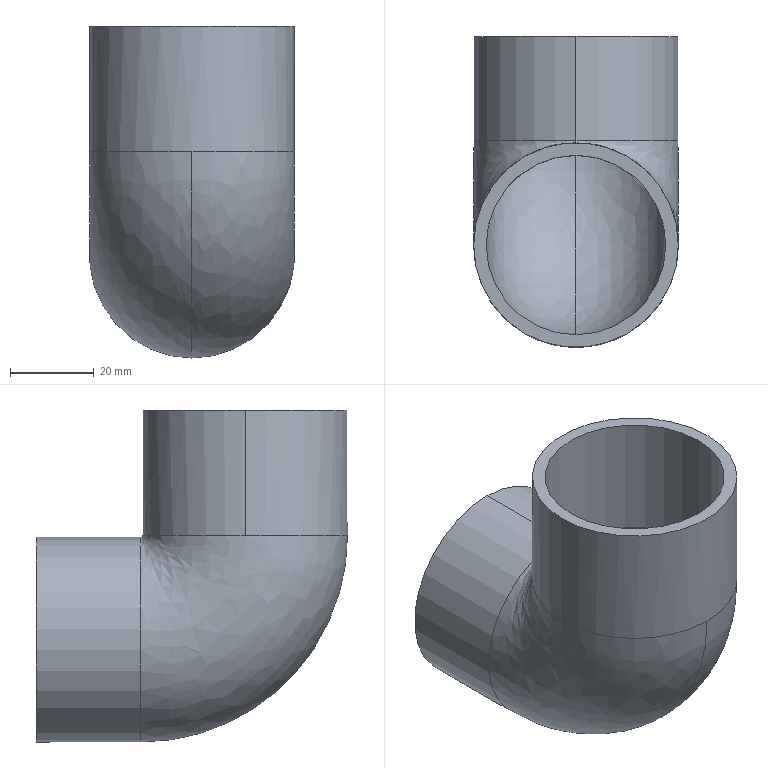Component | SolidWorks | YC1-250-04BalancerAssembly#16673-1_Rc11-4Elbow-1 | 1 solid | 14 faces | box 49 x 74.5 x 79.5 mm | volume 40870 mm3 | cylinder 8 | spline 4 | plane 2 | commonest cylinder face diameters 49 x4 43 x4 | material Plain Carbon Steel
STEP:
#1=COLOUR_RGB('',0.7922,0.8196,0.9333);
#2=FILL_AREA_STYLE_COLOUR('',#1);
#3=FILL_AREA_STYLE('',(#2));
#4=SURFACE_STYLE_FILL_AREA(#3);
#5=SURFACE_SIDE_STYLE('',(#4));
#6=SURFACE_STYLE_USAGE(.BOTH.,#5);
#7=PRESENTATION_STYLE_ASSIGNMENT((#6));
#8=CARTESIAN_POINT('',(-19.075,156.398,-8.524));
#9=VERTEX_POINT('',#8);
#10=CARTESIAN_POINT('',(-18.11,157.362,-8.524));
#11=VERTEX_POINT('',#10);
#12=CARTESIAN_POINT('',(-18.11,156.398,-8.524));
#13=DIRECTION('',(-0.,-0.,-1.));
#14=DIRECTION('',(0.,-1.,0.));
#15=AXIS2_PLACEMENT_3D('',#12,#13,#14);
#16=CIRCLE('',#15,0.9646);
#17=EDGE_CURVE('',#9,#11,#16,.T.);
#18=ORIENTED_EDGE('',*,*,#17,.T.);
#19=CARTESIAN_POINT('',(-18.11,157.382,-8.543));
#20=VERTEX_POINT('',#19);
#21=CARTESIAN_POINT('',(-18.11,157.382,-8.524));
#22=DIRECTION('',(1.,0.,-0.));
#23=DIRECTION('',(0.,0.,-1.));
#24=AXIS2_PLACEMENT_3D('',#21,#22,#23);
#25=CIRCLE('',#24,0.01969);
#26=EDGE_CURVE('',#11,#20,#25,.T.);
#27=ORIENTED_EDGE('',*,*,#26,.T.);
#28=CARTESIAN_POINT('',(-18.11,157.382,-10.472));
#29=VERTEX_POINT('',#28);
#30=CARTESIAN_POINT('',(-18.11,157.382,-9.508));
#31=DIRECTION('',(0.,-1.,0.));
#32=DIRECTION('',(0.,0.,-1.));
#33=AXIS2_PLACEMENT_3D('',#30,#31,#32);
#34=CIRCLE('',#33,0.9646);
#35=EDGE_CURVE('',#20,#29,#34,.T.);
#36=ORIENTED_EDGE('',*,*,#35,.T.);
#37=CARTESIAN_POINT('',(-18.11,155.433,-8.524));
#38=VERTEX_POINT('',#37);
#39=CARTESIAN_POINT('',(-18.11,157.382,-8.524));
#40=DIRECTION('',(1.,0.,-0.));
#41=DIRECTION('',(0.,0.,-1.));
#42=AXIS2_PLACEMENT_3D('',#39,#40,#41);
#43=CIRCLE('',#42,1.949);
#44=EDGE_CURVE('',#38,#29,#43,.T.);
#45=ORIENTED_EDGE('',*,*,#44,.F.);
#46=CARTESIAN_POINT('',(-18.11,156.398,-8.524));
#47=DIRECTION('',(-0.,-0.,-1.));
#48=DIRECTION('',(0.,-1.,0.));
#49=AXIS2_PLACEMENT_3D('',#46,#47,#48);
#50=CIRCLE('',#49,0.9646);
#51=EDGE_CURVE('',#38,#9,#50,.T.);
#52=ORIENTED_EDGE('',*,*,#51,.T.);
#53=EDGE_LOOP('',(#18,#27,#36,#45,#52));
#54=FACE_OUTER_BOUND('',#53,.T.);
#55=CARTESIAN_POINT('',(-18.11,155.433,-8.524));
#56=CARTESIAN_POINT('',(-18.11,155.433,-9.665));
#57=CARTESIAN_POINT('',(-18.11,156.24,-10.472));
#58=CARTESIAN_POINT('',(-18.11,157.382,-10.472));
#59=CARTESIAN_POINT('',(-20.039,155.433,-8.524));
#60=CARTESIAN_POINT('',(-20.039,155.433,-9.665));
#61=CARTESIAN_POINT('',(-20.039,156.24,-10.472));
#62=CARTESIAN_POINT('',(-20.039,157.382,-10.472));
#63=CARTESIAN_POINT('',(-20.039,157.362,-8.524));
#64=CARTESIAN_POINT('',(-20.039,157.362,-8.535));
#65=CARTESIAN_POINT('',(-20.039,157.37,-8.543));
#66=CARTESIAN_POINT('',(-20.039,157.382,-8.543));
#67=CARTESIAN_POINT('',(-18.11,157.362,-8.524));
#68=CARTESIAN_POINT('',(-18.11,157.362,-8.535));
#69=CARTESIAN_POINT('',(-18.11,157.37,-8.543));
#70=CARTESIAN_POINT('',(-18.11,157.382,-8.543));
#71=(BOUNDED_SURFACE()B_SPLINE_SURFACE(3,3,((#55,#56,#57,#58),(#59,#60,#61,#62),(#63,#64,#65,#66),(#67,#68,#69,#70)),.UNSPECIFIED.,.F.,.F.,.F.)B_SPLINE_SURFACE_WITH_KNOTS((4,4),(4,4),(0.,1.),(0.,1.),.UNSPECIFIED.)GEOMETRIC_REPRESENTATION_ITEM()RATIONAL_B_SPLINE_SURFACE(((1.,0.8047,0.8047,1.),(0.3333,0.2682,0.2682,0.3333),(0.3333,0.2682,0.2682,0.3333),(1.,0.8047,0.8047,1.)))REPRESENTATION_ITEM('')SURFACE());
#72=ADVANCED_FACE('',(#54),#71,.T.);
#73=CARTESIAN_POINT('',(-18.11,157.382,-9.508));
#74=DIRECTION('',(0.,-1.,0.));
#75=DIRECTION('',(0.,0.,-1.));
#76=AXIS2_PLACEMENT_3D('',#73,#74,#75);
#77=CIRCLE('',#76,0.9646);
#78=EDGE_CURVE('',#29,#20,#77,.T.);
#79=ORIENTED_EDGE('',*,*,#78,.F.);
#80=CARTESIAN_POINT('',(-18.11,158.366,-10.472));
#81=VERTEX_POINT('',#80);
#82=CARTESIAN_POINT('',(-18.11,157.382,-10.472));
#83=DIRECTION('',(0.,1.,-0.));
#84=VECTOR('',#83,39.37);
#85=LINE('',#82,#84);
#86=EDGE_CURVE('',#29,#81,#85,.T.);
#87=ORIENTED_EDGE('',*,*,#86,.T.);
#88=CARTESIAN_POINT('',(-18.11,158.366,-8.543));
#89=VERTEX_POINT('',#88);
#90=CARTESIAN_POINT('',(-18.11,158.366,-9.508));
#91=DIRECTION('',(-0.,-1.,0.));
#92=DIRECTION('',(0.,0.,1.));
#93=AXIS2_PLACEMENT_3D('',#90,#91,#92);
#94=CIRCLE('',#93,0.9646);
#95=EDGE_CURVE('',#81,#89,#94,.T.);
#96=ORIENTED_EDGE('',*,*,#95,.T.);
#97=CARTESIAN_POINT('',(-18.11,157.382,-8.543));
#98=DIRECTION('',(0.,1.,-0.));
#99=VECTOR('',#98,39.37);
#100=LINE('',#97,#99);
#101=EDGE_CURVE('',#20,#89,#100,.T.);
#102=ORIENTED_EDGE('',*,*,#101,.F.);
#103=EDGE_LOOP('',(#79,#87,#96,#102));
#104=FACE_OUTER_BOUND('',#103,.T.);
#105=CARTESIAN_POINT('',(-18.11,157.382,-9.508));
#106=DIRECTION('',(0.,1.,-0.));
#107=DIRECTION('',(0.,0.,1.));
#108=AXIS2_PLACEMENT_3D('',#105,#106,#107);
#109=CYLINDRICAL_SURFACE('',#108,0.9646);
#110=ADVANCED_FACE('',(#104),#109,.T.);
#111=ORIENTED_EDGE('',*,*,#17,.F.);
#112=CARTESIAN_POINT('',(-19.075,156.398,-7.343));
#113=VERTEX_POINT('',#112);
#114=CARTESIAN_POINT('',(-19.075,156.398,-8.524));
#115=DIRECTION('',(0.,0.,1.));
#116=VECTOR('',#115,39.37);
#117=LINE('',#114,#116);
#118=EDGE_CURVE('',#9,#113,#117,.T.);
#119=ORIENTED_EDGE('',*,*,#118,.T.);
#120=CARTESIAN_POINT('',(-17.146,156.398,-7.343));
#121=VERTEX_POINT('',#120);
#122=CARTESIAN_POINT('',(-18.11,156.398,-7.343));
#123=DIRECTION('',(-0.,-0.,-1.));
#124=DIRECTION('',(1.,0.,0.));
#125=AXIS2_PLACEMENT_3D('',#122,#123,#124);
#126=CIRCLE('',#125,0.9646);
#127=EDGE_CURVE('',#113,#121,#126,.T.);
#128=ORIENTED_EDGE('',*,*,#127,.T.);
#129=CARTESIAN_POINT('',(-17.146,156.398,-8.524));
#130=VERTEX_POINT('',#129);
#131=CARTESIAN_POINT('',(-17.146,156.398,-8.524));
#132=DIRECTION('',(0.,0.,1.));
#133=VECTOR('',#132,39.37);
#134=LINE('',#131,#133);
#135=EDGE_CURVE('',#130,#121,#134,.T.);
#136=ORIENTED_EDGE('',*,*,#135,.F.);
#137=CARTESIAN_POINT('',(-18.11,156.398,-8.524));
#138=DIRECTION('',(-0.,-0.,-1.));
#139=DIRECTION('',(0.,-1.,0.));
#140=AXIS2_PLACEMENT_3D('',#137,#138,#139);
#141=CIRCLE('',#140,0.9646);
#142=EDGE_CURVE('',#11,#130,#141,.T.);
#143=ORIENTED_EDGE('',*,*,#142,.F.);
#144=EDGE_LOOP('',(#111,#119,#128,#136,#143));
#145=FACE_OUTER_BOUND('',#144,.T.);
#146=CARTESIAN_POINT('',(-18.11,156.398,-8.524));
#147=DIRECTION('',(0.,0.,1.));
#148=DIRECTION('',(1.,0.,0.));
#149=AXIS2_PLACEMENT_3D('',#146,#147,#148);
#150=CYLINDRICAL_SURFACE('',#149,0.9646);
#151=ADVANCED_FACE('',(#145),#150,.T.);
#152=CARTESIAN_POINT('',(-18.11,157.382,-10.354));
#153=VERTEX_POINT('',#152);
#154=CARTESIAN_POINT('',(-18.11,157.382,-8.661));
#155=VERTEX_POINT('',#154);
#156=CARTESIAN_POINT('',(-18.11,157.382,-9.508));
#157=DIRECTION('',(0.,1.,-0.));
#158=DIRECTION('',(0.,0.,1.));
#159=AXIS2_PLACEMENT_3D('',#156,#157,#158);
#160=CIRCLE('',#159,0.8465);
#161=EDGE_CURVE('',#153,#155,#160,.T.);
#162=ORIENTED_EDGE('',*,*,#161,.F.);
#163=CARTESIAN_POINT('',(-18.11,158.366,-10.354));
#164=VERTEX_POINT('',#163);
#165=CARTESIAN_POINT('',(-18.11,157.382,-10.354));
#166=DIRECTION('',(0.,1.,-0.));
#167=VECTOR('',#166,39.37);
#168=LINE('',#165,#167);
#169=EDGE_CURVE('',#153,#164,#168,.T.);
#170=ORIENTED_EDGE('',*,*,#169,.T.);
#171=CARTESIAN_POINT('',(-18.11,158.366,-8.661));
#172=VERTEX_POINT('',#171);
#173=CARTESIAN_POINT('',(-18.11,158.366,-9.508));
#174=DIRECTION('',(-0.,-1.,0.));
#175=DIRECTION('',(0.,0.,1.));
#176=AXIS2_PLACEMENT_3D('',#173,#174,#175);
#177=CIRCLE('',#176,0.8465);
#178=EDGE_CURVE('',#172,#164,#177,.T.);
#179=ORIENTED_EDGE('',*,*,#178,.F.);
#180=CARTESIAN_POINT('',(-18.11,157.382,-8.661));
#181=DIRECTION('',(0.,1.,-0.));
#182=VECTOR('',#181,39.37);
#183=LINE('',#180,#182);
#184=EDGE_CURVE('',#155,#172,#183,.T.);
#185=ORIENTED_EDGE('',*,*,#184,.F.);
#186=EDGE_LOOP('',(#162,#170,#179,#185));
#187=FACE_OUTER_BOUND('',#186,.T.);
#188=CARTESIAN_POINT('',(-18.11,157.382,-9.508));
#189=DIRECTION('',(0.,1.,-0.));
#190=DIRECTION('',(0.,0.,1.));
#191=AXIS2_PLACEMENT_3D('',#188,#189,#190);
#192=CYLINDRICAL_SURFACE('',#191,0.8465);
#193=ADVANCED_FACE('',(#187),#192,.F.);
#194=CARTESIAN_POINT('',(-18.957,156.398,-8.524));
#195=VERTEX_POINT('',#194);
#196=CARTESIAN_POINT('',(-18.11,155.551,-8.524));
#197=VERTEX_POINT('',#196);
#198=CARTESIAN_POINT('',(-18.11,156.398,-8.524));
#199=DIRECTION('',(0.,0.,1.));
#200=DIRECTION('',(1.,0.,0.));
#201=AXIS2_PLACEMENT_3D('',#198,#199,#200);
#202=CIRCLE('',#201,0.8465);
#203=EDGE_CURVE('',#195,#197,#202,.T.);
#204=ORIENTED_EDGE('',*,*,#203,.F.);
#205=CARTESIAN_POINT('',(-18.957,156.398,-7.343));
#206=VERTEX_POINT('',#205);
#207=CARTESIAN_POINT('',(-18.957,156.398,-8.524));
#208=DIRECTION('',(0.,0.,1.));
#209=VECTOR('',#208,39.37);
#210=LINE('',#207,#209);
#211=EDGE_CURVE('',#195,#206,#210,.T.);
#212=ORIENTED_EDGE('',*,*,#211,.T.);
#213=CARTESIAN_POINT('',(-17.264,156.398,-7.343));
#214=VERTEX_POINT('',#213);
#215=CARTESIAN_POINT('',(-18.11,156.398,-7.343));
#216=DIRECTION('',(0.,0.,1.));
#217=DIRECTION('',(1.,0.,0.));
#218=AXIS2_PLACEMENT_3D('',#215,#216,#217);
#219=CIRCLE('',#218,0.8465);
#220=EDGE_CURVE('',#206,#214,#219,.T.);
#221=ORIENTED_EDGE('',*,*,#220,.T.);
#222=CARTESIAN_POINT('',(-17.264,156.398,-8.524));
#223=VERTEX_POINT('',#222);
#224=CARTESIAN_POINT('',(-17.264,156.398,-8.524));
#225=DIRECTION('',(0.,0.,1.));
#226=VECTOR('',#225,39.37);
#227=LINE('',#224,#226);
#228=EDGE_CURVE('',#223,#214,#227,.T.);
#229=ORIENTED_EDGE('',*,*,#228,.F.);
#230=CARTESIAN_POINT('',(-18.11,156.398,-8.524));
#231=DIRECTION('',(0.,0.,1.));
#232=DIRECTION('',(1.,0.,0.));
#233=AXIS2_PLACEMENT_3D('',#230,#231,#232);
#234=CIRCLE('',#233,0.8465);
#235=EDGE_CURVE('',#197,#223,#234,.T.);
#236=ORIENTED_EDGE('',*,*,#235,.F.);
#237=EDGE_LOOP('',(#204,#212,#221,#229,#236));
#238=FACE_OUTER_BOUND('',#237,.T.);
#239=CARTESIAN_POINT('',(-18.11,156.398,-8.524));
#240=DIRECTION('',(0.,0.,1.));
#241=DIRECTION('',(1.,0.,0.));
#242=AXIS2_PLACEMENT_3D('',#239,#240,#241);
#243=CYLINDRICAL_SURFACE('',#242,0.8465);
#244=ADVANCED_FACE('',(#238),#243,.F.);
#245=ORIENTED_EDGE('',*,*,#235,.T.);
#246=CARTESIAN_POINT('',(-18.11,157.244,-8.524));
#247=VERTEX_POINT('',#246);
#248=CARTESIAN_POINT('',(-18.11,156.398,-8.524));
#249=DIRECTION('',(0.,0.,1.));
#250=DIRECTION('',(1.,0.,0.));
#251=AXIS2_PLACEMENT_3D('',#248,#249,#250);
#252=CIRCLE('',#251,0.8465);
#253=EDGE_CURVE('',#223,#247,#252,.T.);
#254=ORIENTED_EDGE('',*,*,#253,.T.);
#255=CARTESIAN_POINT('',(-18.11,157.382,-8.524));
#256=DIRECTION('',(1.,0.,-0.));
#257=DIRECTION('',(0.,0.,-1.));
#258=AXIS2_PLACEMENT_3D('',#255,#256,#257);
#259=CIRCLE('',#258,0.1378);
#260=EDGE_CURVE('',#247,#155,#259,.T.);
#261=ORIENTED_EDGE('',*,*,#260,.T.);
#262=CARTESIAN_POINT('',(-18.11,157.382,-9.508));
#263=DIRECTION('',(0.,1.,-0.));
#264=DIRECTION('',(0.,0.,1.));
#265=AXIS2_PLACEMENT_3D('',#262,#263,#264);
#266=CIRCLE('',#265,0.8465);
#267=EDGE_CURVE('',#155,#153,#266,.T.);
#268=ORIENTED_EDGE('',*,*,#267,.T.);
#269=CARTESIAN_POINT('',(-18.11,157.382,-8.524));
#270=DIRECTION('',(1.,0.,-0.));
#271=DIRECTION('',(0.,0.,-1.));
#272=AXIS2_PLACEMENT_3D('',#269,#270,#271);
#273=CIRCLE('',#272,1.831);
#274=EDGE_CURVE('',#197,#153,#273,.T.);
#275=ORIENTED_EDGE('',*,*,#274,.F.);
#276=EDGE_LOOP('',(#245,#254,#261,#268,#275));
#277=FACE_OUTER_BOUND('',#276,.T.);
#278=CARTESIAN_POINT('',(-18.11,157.244,-8.524));
#279=CARTESIAN_POINT('',(-18.11,157.244,-8.604));
#280=CARTESIAN_POINT('',(-18.11,157.301,-8.661));
#281=CARTESIAN_POINT('',(-18.11,157.382,-8.661));
#282=CARTESIAN_POINT('',(-16.417,157.244,-8.524));
#283=CARTESIAN_POINT('',(-16.417,157.244,-8.604));
#284=CARTESIAN_POINT('',(-16.417,157.301,-8.661));
#285=CARTESIAN_POINT('',(-16.417,157.382,-8.661));
#286=CARTESIAN_POINT('',(-16.417,155.551,-8.524));
#287=CARTESIAN_POINT('',(-16.417,155.551,-9.596));
#288=CARTESIAN_POINT('',(-16.417,156.309,-10.354));
#289=CARTESIAN_POINT('',(-16.417,157.382,-10.354));
#290=CARTESIAN_POINT('',(-18.11,155.551,-8.524));
#291=CARTESIAN_POINT('',(-18.11,155.551,-9.596));
#292=CARTESIAN_POINT('',(-18.11,156.309,-10.354));
#293=CARTESIAN_POINT('',(-18.11,157.382,-10.354));
#294=(BOUNDED_SURFACE()B_SPLINE_SURFACE(3,3,((#278,#279,#280,#281),(#282,#283,#284,#285),(#286,#287,#288,#289),(#290,#291,#292,#293)),.UNSPECIFIED.,.F.,.F.,.F.)B_SPLINE_SURFACE_WITH_KNOTS((4,4),(4,4),(0.,1.),(0.,1.),.UNSPECIFIED.)GEOMETRIC_REPRESENTATION_ITEM()RATIONAL_B_SPLINE_SURFACE(((1.,0.8047,0.8047,1.),(0.3333,0.2682,0.2682,0.3333),(0.3333,0.2682,0.2682,0.3333),(1.,0.8047,0.8047,1.)))REPRESENTATION_ITEM('')SURFACE());
#295=ADVANCED_FACE('',(#277),#294,.F.);
#296=ORIENTED_EDGE('',*,*,#26,.F.);
#297=ORIENTED_EDGE('',*,*,#142,.T.);
#298=CARTESIAN_POINT('',(-18.11,156.398,-8.524));
#299=DIRECTION('',(-0.,-0.,-1.));
#300=DIRECTION('',(0.,-1.,0.));
#301=AXIS2_PLACEMENT_3D('',#298,#299,#300);
#302=CIRCLE('',#301,0.9646);
#303=EDGE_CURVE('',#130,#38,#302,.T.);
#304=ORIENTED_EDGE('',*,*,#303,.T.);
#305=ORIENTED_EDGE('',*,*,#44,.T.);
#306=ORIENTED_EDGE('',*,*,#78,.T.);
#307=EDGE_LOOP('',(#296,#297,#304,#305,#306));
#308=FACE_OUTER_BOUND('',#307,.T.);
#309=CARTESIAN_POINT('',(-18.11,157.362,-8.524));
#310=CARTESIAN_POINT('',(-18.11,157.362,-8.535));
#311=CARTESIAN_POINT('',(-18.11,157.37,-8.543));
#312=CARTESIAN_POINT('',(-18.11,157.382,-8.543));
#313=CARTESIAN_POINT('',(-16.181,157.362,-8.524));
#314=CARTESIAN_POINT('',(-16.181,157.362,-8.535));
#315=CARTESIAN_POINT('',(-16.181,157.37,-8.543));
#316=CARTESIAN_POINT('',(-16.181,157.382,-8.543));
#317=CARTESIAN_POINT('',(-16.181,155.433,-8.524));
#318=CARTESIAN_POINT('',(-16.181,155.433,-9.665));
#319=CARTESIAN_POINT('',(-16.181,156.24,-10.472));
#320=CARTESIAN_POINT('',(-16.181,157.382,-10.472));
#321=CARTESIAN_POINT('',(-18.11,155.433,-8.524));
#322=CARTESIAN_POINT('',(-18.11,155.433,-9.665));
#323=CARTESIAN_POINT('',(-18.11,156.24,-10.472));
#324=CARTESIAN_POINT('',(-18.11,157.382,-10.472));
#325=(BOUNDED_SURFACE()B_SPLINE_SURFACE(3,3,((#309,#310,#311,#312),(#313,#314,#315,#316),(#317,#318,#319,#320),(#321,#322,#323,#324)),.UNSPECIFIED.,.F.,.F.,.F.)B_SPLINE_SURFACE_WITH_KNOTS((4,4),(4,4),(0.,1.),(0.,1.),.UNSPECIFIED.)GEOMETRIC_REPRESENTATION_ITEM()RATIONAL_B_SPLINE_SURFACE(((1.,0.8047,0.8047,1.),(0.3333,0.2682,0.2682,0.3333),(0.3333,0.2682,0.2682,0.3333),(1.,0.8047,0.8047,1.)))REPRESENTATION_ITEM('')SURFACE());
#326=ADVANCED_FACE('',(#308),#325,.T.);
#327=ORIENTED_EDGE('',*,*,#86,.F.);
#328=ORIENTED_EDGE('',*,*,#35,.F.);
#329=ORIENTED_EDGE('',*,*,#101,.T.);
#330=CARTESIAN_POINT('',(-18.11,158.366,-9.508));
#331=DIRECTION('',(-0.,-1.,0.));
#332=DIRECTION('',(0.,0.,1.));
#333=AXIS2_PLACEMENT_3D('',#330,#331,#332);
#334=CIRCLE('',#333,0.9646);
#335=EDGE_CURVE('',#89,#81,#334,.T.);
#336=ORIENTED_EDGE('',*,*,#335,.T.);
#337=EDGE_LOOP('',(#327,#328,#329,#336));
#338=FACE_OUTER_BOUND('',#337,.T.);
#339=CARTESIAN_POINT('',(-18.11,157.382,-9.508));
#340=DIRECTION('',(0.,1.,-0.));
#341=DIRECTION('',(0.,0.,1.));
#342=AXIS2_PLACEMENT_3D('',#339,#340,#341);
#343=CYLINDRICAL_SURFACE('',#342,0.9646);
#344=ADVANCED_FACE('',(#338),#343,.T.);
#345=ORIENTED_EDGE('',*,*,#118,.F.);
#346=ORIENTED_EDGE('',*,*,#51,.F.);
#347=ORIENTED_EDGE('',*,*,#303,.F.);
#348=ORIENTED_EDGE('',*,*,#135,.T.);
#349=CARTESIAN_POINT('',(-18.11,156.398,-7.343));
#350=DIRECTION('',(-0.,-0.,-1.));
#351=DIRECTION('',(1.,0.,0.));
#352=AXIS2_PLACEMENT_3D('',#349,#350,#351);
#353=CIRCLE('',#352,0.9646);
#354=EDGE_CURVE('',#121,#113,#353,.T.);
#355=ORIENTED_EDGE('',*,*,#354,.T.);
#356=EDGE_LOOP('',(#345,#346,#347,#348,#355));
#357=FACE_OUTER_BOUND('',#356,.T.);
#358=CARTESIAN_POINT('',(-18.11,156.398,-8.524));
#359=DIRECTION('',(0.,0.,1.));
#360=DIRECTION('',(1.,0.,0.));
#361=AXIS2_PLACEMENT_3D('',#358,#359,#360);
#362=CYLINDRICAL_SURFACE('',#361,0.9646);
#363=ADVANCED_FACE('',(#357),#362,.T.);
#364=ORIENTED_EDGE('',*,*,#335,.F.);
#365=ORIENTED_EDGE('',*,*,#95,.F.);
#366=EDGE_LOOP('',(#364,#365));
#367=FACE_OUTER_BOUND('',#366,.T.);
#368=ORIENTED_EDGE('',*,*,#178,.T.);
#369=CARTESIAN_POINT('',(-18.11,158.366,-9.508));
#370=DIRECTION('',(-0.,-1.,0.));
#371=DIRECTION('',(0.,0.,1.));
#372=AXIS2_PLACEMENT_3D('',#369,#370,#371);
#373=CIRCLE('',#372,0.8465);
#374=EDGE_CURVE('',#164,#172,#373,.T.);
#375=ORIENTED_EDGE('',*,*,#374,.T.);
#376=EDGE_LOOP('',(#368,#375));
#377=FACE_BOUND('',#376,.T.);
#378=CARTESIAN_POINT('',(-18.11,158.366,-9.508));
#379=DIRECTION('',(-0.,1.,-0.));
#380=DIRECTION('',(0.,0.,1.));
#381=AXIS2_PLACEMENT_3D('',#378,#379,#380);
#382=PLANE('',#381);
#383=ADVANCED_FACE('',(#367,#377),#382,.T.);
#384=ORIENTED_EDGE('',*,*,#354,.F.);
#385=ORIENTED_EDGE('',*,*,#127,.F.);
#386=EDGE_LOOP('',(#384,#385));
#387=FACE_OUTER_BOUND('',#386,.T.);
#388=CARTESIAN_POINT('',(-18.11,156.398,-7.343));
#389=DIRECTION('',(0.,0.,1.));
#390=DIRECTION('',(1.,0.,0.));
#391=AXIS2_PLACEMENT_3D('',#388,#389,#390);
#392=CIRCLE('',#391,0.8465);
#393=EDGE_CURVE('',#214,#206,#392,.T.);
#394=ORIENTED_EDGE('',*,*,#393,.F.);
#395=ORIENTED_EDGE('',*,*,#220,.F.);
#396=EDGE_LOOP('',(#394,#395));
#397=FACE_BOUND('',#396,.T.);
#398=CARTESIAN_POINT('',(-18.11,156.398,-7.343));
#399=DIRECTION('',(-0.,-0.,-1.));
#400=DIRECTION('',(-1.,0.,0.));
#401=AXIS2_PLACEMENT_3D('',#398,#399,#400);
#402=PLANE('',#401);
#403=ADVANCED_FACE('',(#387,#397),#402,.F.);
#404=ORIENTED_EDGE('',*,*,#169,.F.);
#405=ORIENTED_EDGE('',*,*,#267,.F.);
#406=ORIENTED_EDGE('',*,*,#184,.T.);
#407=ORIENTED_EDGE('',*,*,#374,.F.);
#408=EDGE_LOOP('',(#404,#405,#406,#407));
#409=FACE_OUTER_BOUND('',#408,.T.);
#410=CARTESIAN_POINT('',(-18.11,157.382,-9.508));
#411=DIRECTION('',(0.,1.,-0.));
#412=DIRECTION('',(0.,0.,1.));
#413=AXIS2_PLACEMENT_3D('',#410,#411,#412);
#414=CYLINDRICAL_SURFACE('',#413,0.8465);
#415=ADVANCED_FACE('',(#409),#414,.F.);
#416=ORIENTED_EDGE('',*,*,#211,.F.);
#417=CARTESIAN_POINT('',(-18.11,156.398,-8.524));
#418=DIRECTION('',(0.,0.,1.));
#419=DIRECTION('',(1.,0.,0.));
#420=AXIS2_PLACEMENT_3D('',#417,#418,#419);
#421=CIRCLE('',#420,0.8465);
#422=EDGE_CURVE('',#247,#195,#421,.T.);
#423=ORIENTED_EDGE('',*,*,#422,.F.);
#424=ORIENTED_EDGE('',*,*,#253,.F.);
#425=ORIENTED_EDGE('',*,*,#228,.T.);
#426=ORIENTED_EDGE('',*,*,#393,.T.);
#427=EDGE_LOOP('',(#416,#423,#424,#425,#426));
#428=FACE_OUTER_BOUND('',#427,.T.);
#429=CARTESIAN_POINT('',(-18.11,156.398,-8.524));
#430=DIRECTION('',(0.,0.,1.));
#431=DIRECTION('',(1.,0.,0.));
#432=AXIS2_PLACEMENT_3D('',#429,#430,#431);
#433=CYLINDRICAL_SURFACE('',#432,0.8465);
#434=ADVANCED_FACE('',(#428),#433,.F.);
#435=ORIENTED_EDGE('',*,*,#260,.F.);
#436=ORIENTED_EDGE('',*,*,#422,.T.);
#437=ORIENTED_EDGE('',*,*,#203,.T.);
#438=ORIENTED_EDGE('',*,*,#274,.T.);
#439=ORIENTED_EDGE('',*,*,#161,.T.);
#440=EDGE_LOOP('',(#435,#436,#437,#438,#439));
#441=FACE_OUTER_BOUND('',#440,.T.);
#442=CARTESIAN_POINT('',(-18.11,155.551,-8.524));
#443=CARTESIAN_POINT('',(-18.11,155.551,-9.596));
#444=CARTESIAN_POINT('',(-18.11,156.309,-10.354));
#445=CARTESIAN_POINT('',(-18.11,157.382,-10.354));
#446=CARTESIAN_POINT('',(-19.803,155.551,-8.524));
#447=CARTESIAN_POINT('',(-19.803,155.551,-9.596));
#448=CARTESIAN_POINT('',(-19.803,156.309,-10.354));
#449=CARTESIAN_POINT('',(-19.803,157.382,-10.354));
#450=CARTESIAN_POINT('',(-19.803,157.244,-8.524));
#451=CARTESIAN_POINT('',(-19.803,157.244,-8.604));
#452=CARTESIAN_POINT('',(-19.803,157.301,-8.661));
#453=CARTESIAN_POINT('',(-19.803,157.382,-8.661));
#454=CARTESIAN_POINT('',(-18.11,157.244,-8.524));
#455=CARTESIAN_POINT('',(-18.11,157.244,-8.604));
#456=CARTESIAN_POINT('',(-18.11,157.301,-8.661));
#457=CARTESIAN_POINT('',(-18.11,157.382,-8.661));
#458=(BOUNDED_SURFACE()B_SPLINE_SURFACE(3,3,((#442,#443,#444,#445),(#446,#447,#448,#449),(#450,#451,#452,#453),(#454,#455,#456,#457)),.UNSPECIFIED.,.F.,.F.,.F.)B_SPLINE_SURFACE_WITH_KNOTS((4,4),(4,4),(0.,1.),(0.,1.),.UNSPECIFIED.)GEOMETRIC_REPRESENTATION_ITEM()RATIONAL_B_SPLINE_SURFACE(((1.,0.8047,0.8047,1.),(0.3333,0.2682,0.2682,0.3333),(0.3333,0.2682,0.2682,0.3333),(1.,0.8047,0.8047,1.)))REPRESENTATION_ITEM('')SURFACE());
#459=ADVANCED_FACE('',(#441),#458,.F.);
#460=CLOSED_SHELL('',(#72,#110,#151,#193,#244,#295,#326,#344,#363,#383,#403,#415,#434,#459));
#461=MANIFOLD_SOLID_BREP('',#460);
#462=STYLED_ITEM('',(#7),#461);
#463=(LENGTH_UNIT()NAMED_UNIT(*)SI_UNIT($,.METRE.));
#464=LENGTH_MEASURE_WITH_UNIT(LENGTH_MEASURE(0.0254),#463);
#465=DIMENSIONAL_EXPONENTS(1.,0.,0.,0.,0.,0.,0.);
#466=(CONVERSION_BASED_UNIT('',#464)LENGTH_UNIT()NAMED_UNIT(#465));
#467=UNCERTAINTY_MEASURE_WITH_UNIT(LENGTH_MEASURE(0.00001),#466,'','');
#468=(NAMED_UNIT(*)PLANE_ANGLE_UNIT()SI_UNIT($,.RADIAN.));
#469=(NAMED_UNIT(*)SI_UNIT($,.STERADIAN.)SOLID_ANGLE_UNIT());
#470=(GEOMETRIC_REPRESENTATION_CONTEXT(3)GLOBAL_UNCERTAINTY_ASSIGNED_CONTEXT((#467))GLOBAL_UNIT_ASSIGNED_CONTEXT((#466,#468,#469))REPRESENTATION_CONTEXT('',''));
#471=MECHANICAL_DESIGN_GEOMETRIC_PRESENTATION_REPRESENTATION('',(#462),#470);
#472=PRESENTATION_LAYER_ASSIGNMENT('','',(#462));
#473=CARTESIAN_POINT('',(0.,0.,0.));
#474=DIRECTION('',(0.,0.,1.));
#475=DIRECTION('',(1.,0.,0.));
#476=AXIS2_PLACEMENT_3D('',#473,#474,#475);
#477=(LENGTH_UNIT()NAMED_UNIT(*)SI_UNIT($,.METRE.));
#478=LENGTH_MEASURE_WITH_UNIT(LENGTH_MEASURE(0.0254),#477);
#479=DIMENSIONAL_EXPONENTS(1.,0.,0.,0.,0.,0.,0.);
#480=(CONVERSION_BASED_UNIT('',#478)LENGTH_UNIT()NAMED_UNIT(#479));
#481=UNCERTAINTY_MEASURE_WITH_UNIT(LENGTH_MEASURE(0.00001),#480,'','');
#482=(NAMED_UNIT(*)PLANE_ANGLE_UNIT()SI_UNIT($,.RADIAN.));
#483=(NAMED_UNIT(*)SI_UNIT($,.STERADIAN.)SOLID_ANGLE_UNIT());
#484=(GEOMETRIC_REPRESENTATION_CONTEXT(3)GLOBAL_UNCERTAINTY_ASSIGNED_CONTEXT((#481))GLOBAL_UNIT_ASSIGNED_CONTEXT((#480,#482,#483))REPRESENTATION_CONTEXT('',''));
#485=ADVANCED_BREP_SHAPE_REPRESENTATION('',(#461,#476),#484);